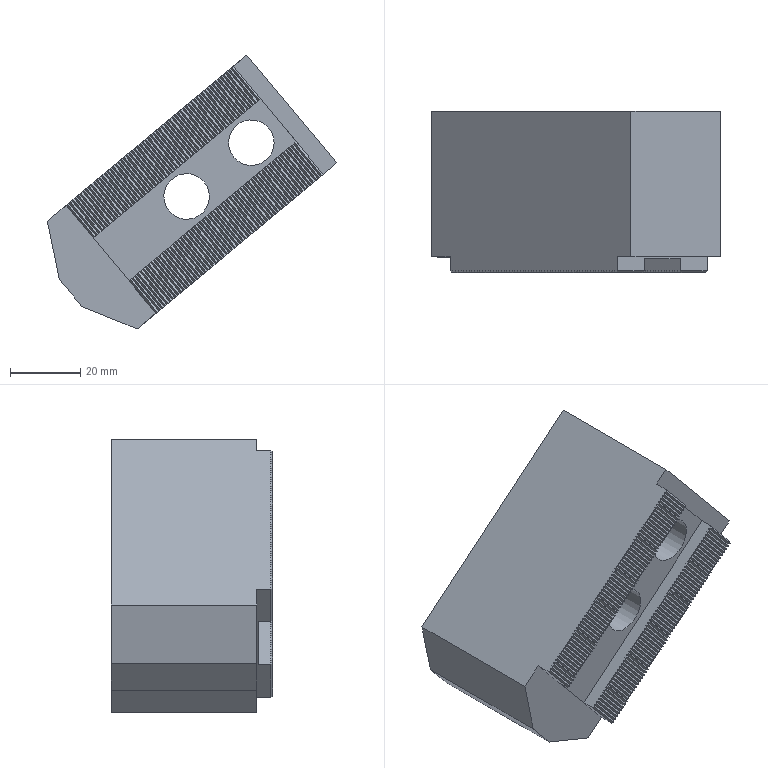Component | SolidWorks | K51-2_K51-4-2 | 1 solid | 272 faces | box 82.48 x 46 x 78.06 mm | volume 119553 mm3 | plane 264 | cylinder 8 | commonest cylinder face diameters 20 x4 13 x4
build123d program:
from build123d import *
from OCP.BRepFilletAPI import BRepFilletAPI_MakeChamfer

# Parameters (mm, degrees)
BOSS_EXTRUDE1_DEPTH                                  = 82
SKETCH2_W                                            = 15
SKETCH2_H                                            = 4.5
SKETCH2_W_2                                          = 5
CUT_EXTRUDE1_DEPTH                                   = 82
COUNTERBORE_HOLE_FOR_M12_HEX_HEAD_BOLT_1_D           = 13
COUNTERBORE_HOLE_FOR_M12_HEX_HEAD_BOLT_1_CBORE_D     = 20
COUNTERBORE_HOLE_FOR_M12_HEX_HEAD_BOLT_1_CBORE_DEPTH = 20
CHAMFER1_SIZE                                        = 8
CHAMFER1_SIZE2                                       = 15
CUT_EXTRUDE2_DEPTH                                   = 82
LPATTERN1_COUNT                                      = 62
LPATTERN1_PITCH                                      = 1


with BuildPart() as part:
    # Sketch1 → Boss-Extrude1 (new body)
    with BuildSketch(Plane.XY):
        Polygon((-20, 42), (20, 42), (20, -4), (8, -4), (8, 0), (-8, 0), (-8, -4), (-20, -4), align=None)
    extrude(amount=BOSS_EXTRUDE1_DEPTH)

    # Sketch2 → Cut-Extrude1 (cut)
    with BuildSketch(Plane(origin=(20, 0, 0), x_dir=(0, 0, -1), z_dir=(1, 0, 0))):
        with Locations((-74.5, -1.75)):
            Rectangle(SKETCH2_W, SKETCH2_H)
        with Locations((-2.5, -1.75)):
            Rectangle(SKETCH2_W_2, SKETCH2_H)
    extrude(amount=-CUT_EXTRUDE1_DEPTH, mode=Mode.SUBTRACT)

    # Counterbore Hole for M12 Hex Head Bolt 1 (through all)
    with Locations(Plane(origin=(0, 42, 15), x_dir=(0, 0, 1), z_dir=(0, 1, 0))):
        with Locations((0, 0), (24, 0)):
            CounterBoreHole(COUNTERBORE_HOLE_FOR_M12_HEX_HEAD_BOLT_1_D / 2, COUNTERBORE_HOLE_FOR_M12_HEX_HEAD_BOLT_1_CBORE_D / 2, COUNTERBORE_HOLE_FOR_M12_HEX_HEAD_BOLT_1_CBORE_DEPTH)

    # Chamfer1: one chamfer whose edges measure the first distance from different faces: ONE call of the kernel's chamfer builder (chamfer() names one face for all edges)
    chamfer1_edges_1 = [part.edges().sort_by_distance(p)[0] for p in [
        (20, 21.25, 82),
    ]]
    chamfer1_side_1 = [part.faces().sort_by_distance(p)[0] for p in [
        (20, 19.507, 40.621),
    ]]
    chamfer1_edges_2 = [part.edges().sort_by_distance(p)[0] for p in [
        (-20, 21.25, 82),
    ]]
    chamfer1_side_2 = [part.faces().sort_by_distance(p)[0] for p in [
        (-20, 19.507, 40.621),
    ]]
    chamfer1 = BRepFilletAPI_MakeChamfer(part.part.solid().wrapped)
    for e in chamfer1_edges_1:
        chamfer1.Add(CHAMFER1_SIZE, CHAMFER1_SIZE2, e.wrapped, chamfer1_side_1[0].wrapped)  # the first distance lies on this face
    for e in chamfer1_edges_2:
        chamfer1.Add(CHAMFER1_SIZE, CHAMFER1_SIZE2, e.wrapped, chamfer1_side_2[0].wrapped)  # the first distance lies on this face
    add(Compound.cast(chamfer1.Shape()), mode=Mode.REPLACE)

    # Sketch7 → Cut-Extrude2 (cut)
    with BuildSketch(Plane.ZY.offset(20)):
        Polygon((4.429, -4.071), (5, -3.5), (5.5, -4), (6, -3.5), (6.5, -4), (6.5, -5.568), (5.5, -5.568), (4.429, -5.568), align=None)
    cut_extrude2 = extrude(amount=-CUT_EXTRUDE2_DEPTH, mode=Mode.SUBTRACT)

    # LPattern1: Cut-Extrude2 ×62
    with Locations(*[(0, 0, i * LPATTERN1_PITCH) for i in range(1, LPATTERN1_COUNT)]):
        add(cut_extrude2, mode=Mode.SUBTRACT)


solid = part.part

# Placed as in the assembly
solid = solid.moved(Location((-275.285, 1010, 60.673), (180, -50.269, -180)))